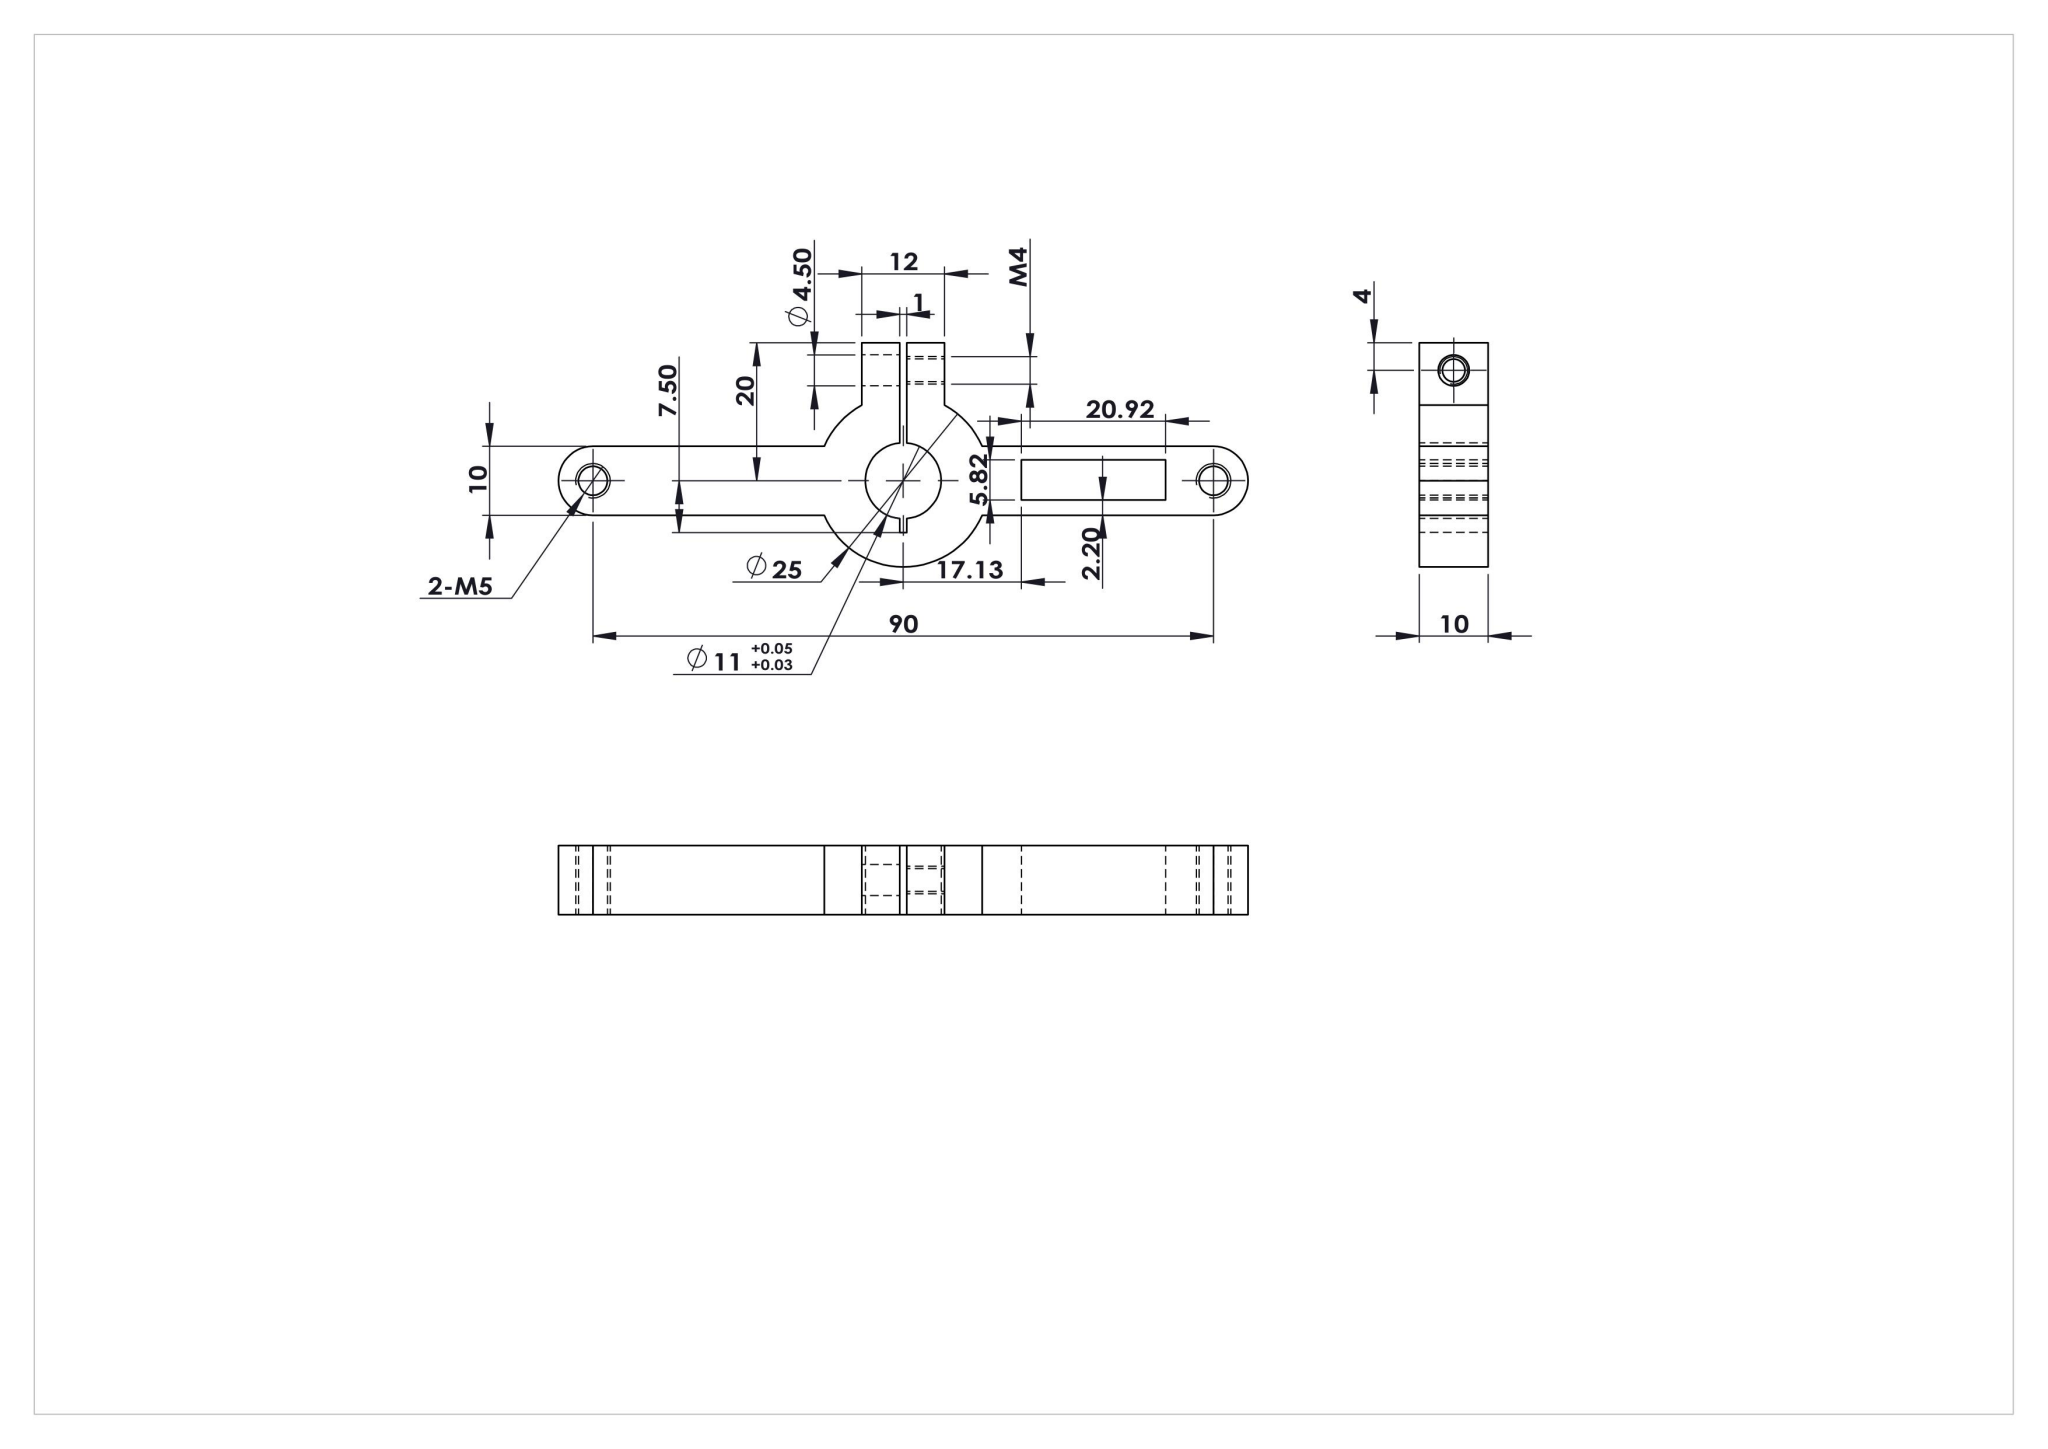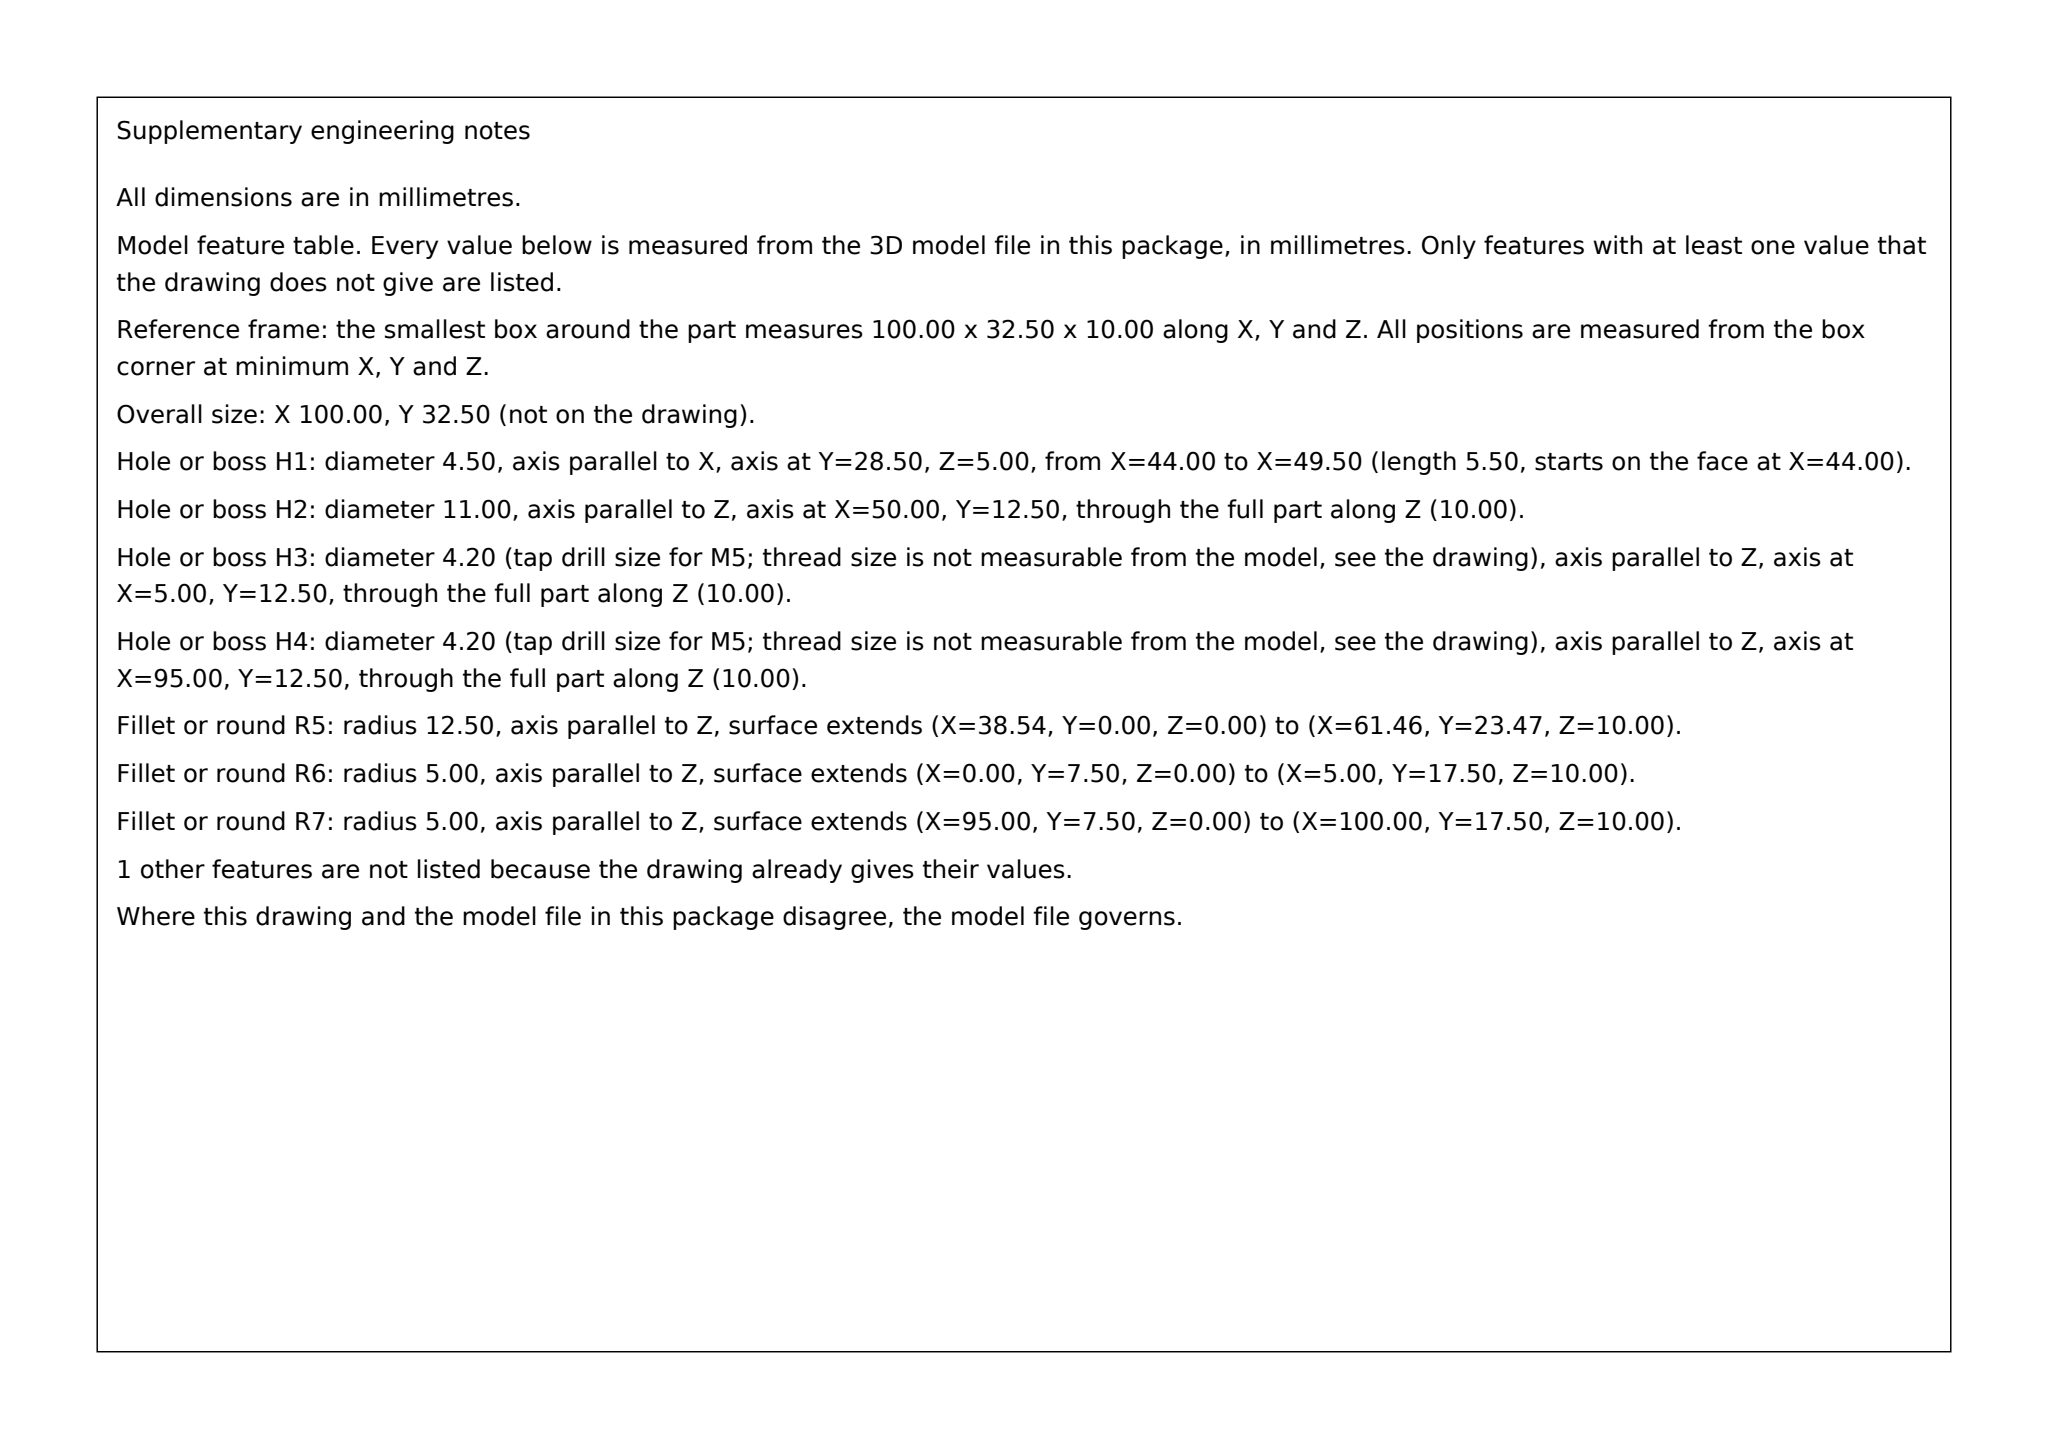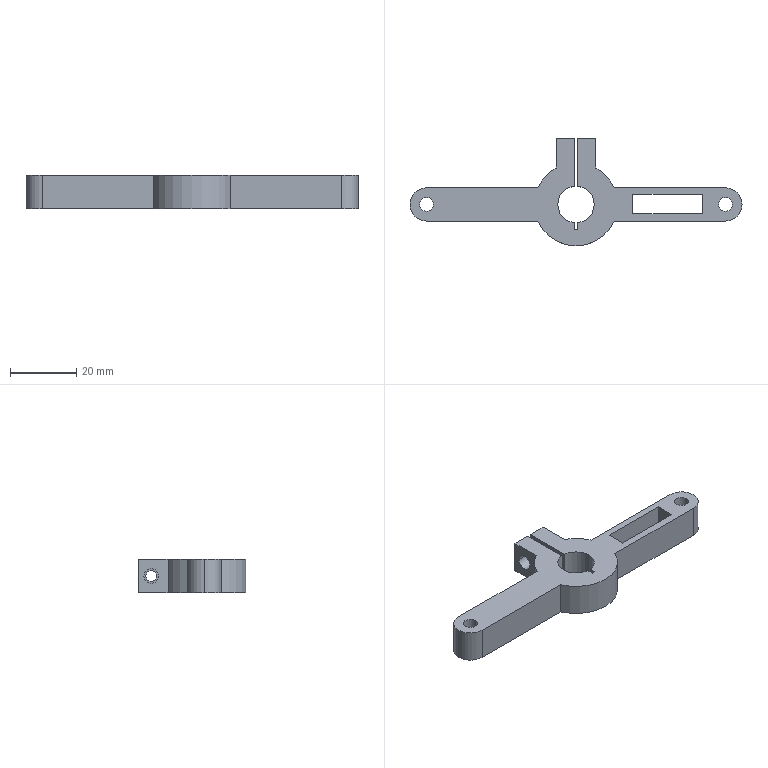Part | SolidWorks | mm | 1 solid | 37 faces | box 100 x 32.5 x 10 mm | volume 10478 mm3 | plane 19 | cylinder 18 | commonest cylinder face diameters 4.2 x4 10 x4 11 x3 25 x3 3.3 x2 4.5 x2